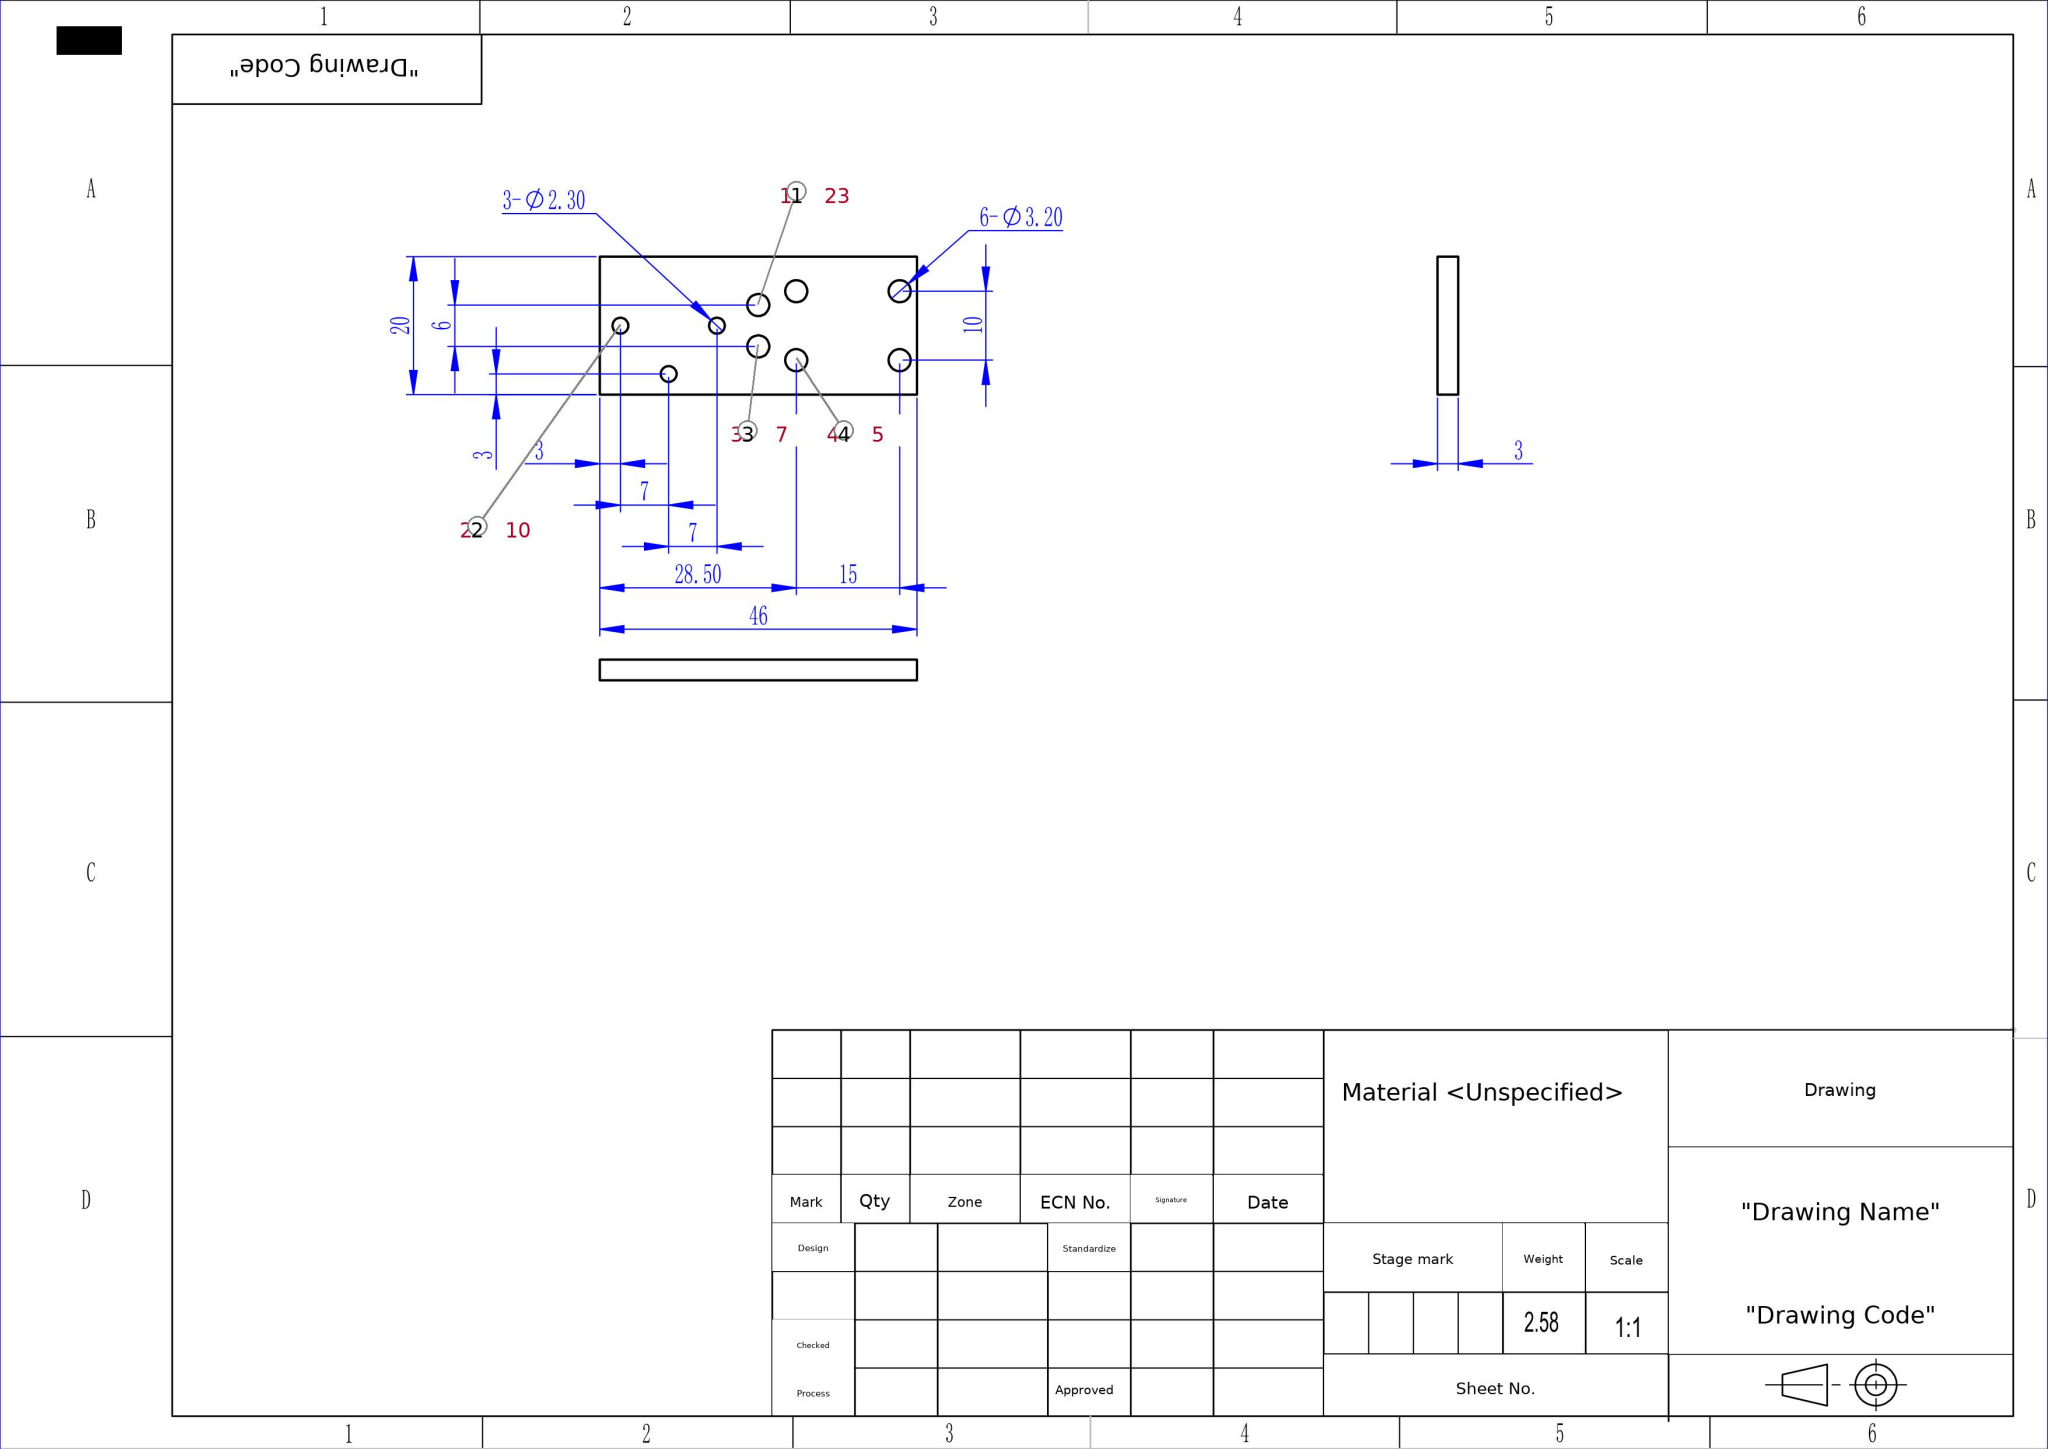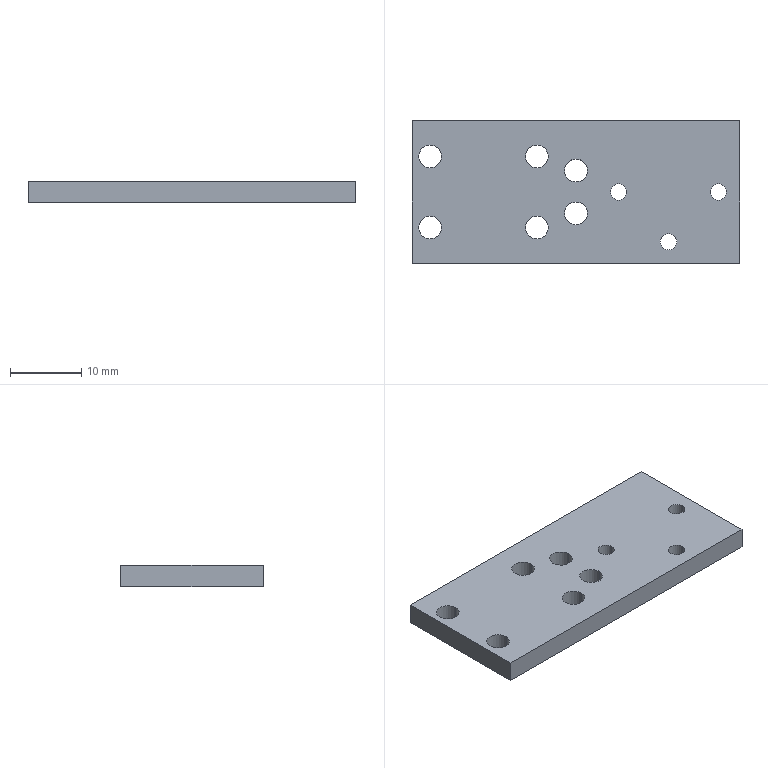Part | SolidWorks | mm | 1 solid | 24 faces | box 46 x 20 x 3 mm | volume 2578 mm3 | cylinder 18 | plane 6 | commonest cylinder face diameters 3.2 x12 2.3 x6
build123d program:
from build123d import *

# Parameters (mm, degrees)
SKETCH1_W           = 46
SKETCH1_H           = 20
SKETCH1_R           = 1.6
SKETCH1_R_2         = 1.15
BOSS_EXTRUDE1_DEPTH = 3


with BuildPart() as part:
    # Sketch1 → Boss-Extrude1 (new body)
    with BuildSketch(Plane.XY):
        with Locations((13, 0)):
            Rectangle(SKETCH1_W, SKETCH1_H)
        with Locations((-7.5, 5)):
            Circle(SKETCH1_R, mode=Mode.SUBTRACT)
        with Locations((7.5, 5)):
            Circle(SKETCH1_R, mode=Mode.SUBTRACT)
        with Locations((7.5, -5)):
            Circle(SKETCH1_R, mode=Mode.SUBTRACT)
        with Locations((-7.5, -5)):
            Circle(SKETCH1_R, mode=Mode.SUBTRACT)
        with Locations((26, -7)):
            Circle(SKETCH1_R_2, mode=Mode.SUBTRACT)
        with Locations((19, 0)):
            Circle(SKETCH1_R_2, mode=Mode.SUBTRACT)
        with Locations((33, 0)):
            Circle(SKETCH1_R_2, mode=Mode.SUBTRACT)
        with Locations((13, 3)):
            Circle(SKETCH1_R, mode=Mode.SUBTRACT)
        with Locations((13, -3)):
            Circle(SKETCH1_R, mode=Mode.SUBTRACT)
    extrude(amount=BOSS_EXTRUDE1_DEPTH)


solid = part.part
STEP:
#1=CARTESIAN_POINT('',(17.85,0.,3.));
#2=VERTEX_POINT('',#1);
#3=CARTESIAN_POINT('',(20.15,0.,3.));
#4=VERTEX_POINT('',#3);
#5=CARTESIAN_POINT('',(19.,0.,3.));
#6=DIRECTION('',(0.,0.,1.));
#7=DIRECTION('',(1.,0.,0.));
#8=AXIS2_PLACEMENT_3D('',#5,#6,#7);
#9=CIRCLE('',#8,1.15);
#10=EDGE_CURVE('',#2,#4,#9,.T.);
#11=ORIENTED_EDGE('',*,*,#10,.T.);
#12=CARTESIAN_POINT('',(20.15,0.,0.));
#13=VERTEX_POINT('',#12);
#14=CARTESIAN_POINT('',(20.15,0.,3.));
#15=DIRECTION('',(0.,0.,-1.));
#16=VECTOR('',#15,1000.);
#17=LINE('',#14,#16);
#18=EDGE_CURVE('',#4,#13,#17,.T.);
#19=ORIENTED_EDGE('',*,*,#18,.T.);
#20=CARTESIAN_POINT('',(17.85,0.,0.));
#21=VERTEX_POINT('',#20);
#22=CARTESIAN_POINT('',(19.,0.,0.));
#23=DIRECTION('',(0.,0.,1.));
#24=DIRECTION('',(1.,0.,0.));
#25=AXIS2_PLACEMENT_3D('',#22,#23,#24);
#26=CIRCLE('',#25,1.15);
#27=EDGE_CURVE('',#21,#13,#26,.T.);
#28=ORIENTED_EDGE('',*,*,#27,.F.);
#29=CARTESIAN_POINT('',(17.85,0.,3.));
#30=DIRECTION('',(0.,0.,-1.));
#31=VECTOR('',#30,1000.);
#32=LINE('',#29,#31);
#33=EDGE_CURVE('',#2,#21,#32,.T.);
#34=ORIENTED_EDGE('',*,*,#33,.F.);
#35=EDGE_LOOP('',(#11,#19,#28,#34));
#36=FACE_OUTER_BOUND('',#35,.T.);
#37=CARTESIAN_POINT('',(19.,0.,3.));
#38=DIRECTION('',(0.,0.,-1.));
#39=DIRECTION('',(-1.,0.,0.));
#40=AXIS2_PLACEMENT_3D('',#37,#38,#39);
#41=CYLINDRICAL_SURFACE('',#40,1.15);
#42=ADVANCED_FACE('',(#36),#41,.F.);
#43=CARTESIAN_POINT('',(24.85,-7.,3.));
#44=VERTEX_POINT('',#43);
#45=CARTESIAN_POINT('',(27.15,-7.,3.));
#46=VERTEX_POINT('',#45);
#47=CARTESIAN_POINT('',(26.,-7.,3.));
#48=DIRECTION('',(0.,0.,1.));
#49=DIRECTION('',(1.,0.,0.));
#50=AXIS2_PLACEMENT_3D('',#47,#48,#49);
#51=CIRCLE('',#50,1.15);
#52=EDGE_CURVE('',#44,#46,#51,.T.);
#53=ORIENTED_EDGE('',*,*,#52,.T.);
#54=CARTESIAN_POINT('',(27.15,-7.,0.));
#55=VERTEX_POINT('',#54);
#56=CARTESIAN_POINT('',(27.15,-7.,3.));
#57=DIRECTION('',(0.,0.,-1.));
#58=VECTOR('',#57,1000.);
#59=LINE('',#56,#58);
#60=EDGE_CURVE('',#46,#55,#59,.T.);
#61=ORIENTED_EDGE('',*,*,#60,.T.);
#62=CARTESIAN_POINT('',(24.85,-7.,0.));
#63=VERTEX_POINT('',#62);
#64=CARTESIAN_POINT('',(26.,-7.,0.));
#65=DIRECTION('',(0.,0.,1.));
#66=DIRECTION('',(1.,0.,0.));
#67=AXIS2_PLACEMENT_3D('',#64,#65,#66);
#68=CIRCLE('',#67,1.15);
#69=EDGE_CURVE('',#63,#55,#68,.T.);
#70=ORIENTED_EDGE('',*,*,#69,.F.);
#71=CARTESIAN_POINT('',(24.85,-7.,3.));
#72=DIRECTION('',(0.,0.,-1.));
#73=VECTOR('',#72,1000.);
#74=LINE('',#71,#73);
#75=EDGE_CURVE('',#44,#63,#74,.T.);
#76=ORIENTED_EDGE('',*,*,#75,.F.);
#77=EDGE_LOOP('',(#53,#61,#70,#76));
#78=FACE_OUTER_BOUND('',#77,.T.);
#79=CARTESIAN_POINT('',(26.,-7.,3.));
#80=DIRECTION('',(0.,0.,-1.));
#81=DIRECTION('',(-1.,0.,0.));
#82=AXIS2_PLACEMENT_3D('',#79,#80,#81);
#83=CYLINDRICAL_SURFACE('',#82,1.15);
#84=ADVANCED_FACE('',(#78),#83,.F.);
#85=CARTESIAN_POINT('',(11.4,-3.,3.));
#86=VERTEX_POINT('',#85);
#87=CARTESIAN_POINT('',(14.6,-3.,3.));
#88=VERTEX_POINT('',#87);
#89=CARTESIAN_POINT('',(13.,-3.,3.));
#90=DIRECTION('',(0.,0.,1.));
#91=DIRECTION('',(1.,0.,0.));
#92=AXIS2_PLACEMENT_3D('',#89,#90,#91);
#93=CIRCLE('',#92,1.6);
#94=EDGE_CURVE('',#86,#88,#93,.T.);
#95=ORIENTED_EDGE('',*,*,#94,.T.);
#96=CARTESIAN_POINT('',(14.6,-3.,0.));
#97=VERTEX_POINT('',#96);
#98=CARTESIAN_POINT('',(14.6,-3.,3.));
#99=DIRECTION('',(0.,0.,-1.));
#100=VECTOR('',#99,1000.);
#101=LINE('',#98,#100);
#102=EDGE_CURVE('',#88,#97,#101,.T.);
#103=ORIENTED_EDGE('',*,*,#102,.T.);
#104=CARTESIAN_POINT('',(11.4,-3.,0.));
#105=VERTEX_POINT('',#104);
#106=CARTESIAN_POINT('',(13.,-3.,0.));
#107=DIRECTION('',(0.,0.,1.));
#108=DIRECTION('',(1.,0.,0.));
#109=AXIS2_PLACEMENT_3D('',#106,#107,#108);
#110=CIRCLE('',#109,1.6);
#111=EDGE_CURVE('',#105,#97,#110,.T.);
#112=ORIENTED_EDGE('',*,*,#111,.F.);
#113=CARTESIAN_POINT('',(11.4,-3.,3.));
#114=DIRECTION('',(0.,0.,-1.));
#115=VECTOR('',#114,1000.);
#116=LINE('',#113,#115);
#117=EDGE_CURVE('',#86,#105,#116,.T.);
#118=ORIENTED_EDGE('',*,*,#117,.F.);
#119=EDGE_LOOP('',(#95,#103,#112,#118));
#120=FACE_OUTER_BOUND('',#119,.T.);
#121=CARTESIAN_POINT('',(13.,-3.,3.));
#122=DIRECTION('',(0.,0.,-1.));
#123=DIRECTION('',(-1.,0.,0.));
#124=AXIS2_PLACEMENT_3D('',#121,#122,#123);
#125=CYLINDRICAL_SURFACE('',#124,1.6);
#126=ADVANCED_FACE('',(#120),#125,.F.);
#127=CARTESIAN_POINT('',(31.85,0.,3.));
#128=VERTEX_POINT('',#127);
#129=CARTESIAN_POINT('',(34.15,0.,3.));
#130=VERTEX_POINT('',#129);
#131=CARTESIAN_POINT('',(33.,0.,3.));
#132=DIRECTION('',(0.,0.,1.));
#133=DIRECTION('',(1.,0.,0.));
#134=AXIS2_PLACEMENT_3D('',#131,#132,#133);
#135=CIRCLE('',#134,1.15);
#136=EDGE_CURVE('',#128,#130,#135,.T.);
#137=ORIENTED_EDGE('',*,*,#136,.T.);
#138=CARTESIAN_POINT('',(34.15,0.,0.));
#139=VERTEX_POINT('',#138);
#140=CARTESIAN_POINT('',(34.15,0.,3.));
#141=DIRECTION('',(0.,0.,-1.));
#142=VECTOR('',#141,1000.);
#143=LINE('',#140,#142);
#144=EDGE_CURVE('',#130,#139,#143,.T.);
#145=ORIENTED_EDGE('',*,*,#144,.T.);
#146=CARTESIAN_POINT('',(31.85,0.,0.));
#147=VERTEX_POINT('',#146);
#148=CARTESIAN_POINT('',(33.,0.,0.));
#149=DIRECTION('',(0.,0.,1.));
#150=DIRECTION('',(1.,0.,0.));
#151=AXIS2_PLACEMENT_3D('',#148,#149,#150);
#152=CIRCLE('',#151,1.15);
#153=EDGE_CURVE('',#147,#139,#152,.T.);
#154=ORIENTED_EDGE('',*,*,#153,.F.);
#155=CARTESIAN_POINT('',(31.85,0.,3.));
#156=DIRECTION('',(0.,0.,-1.));
#157=VECTOR('',#156,1000.);
#158=LINE('',#155,#157);
#159=EDGE_CURVE('',#128,#147,#158,.T.);
#160=ORIENTED_EDGE('',*,*,#159,.F.);
#161=EDGE_LOOP('',(#137,#145,#154,#160));
#162=FACE_OUTER_BOUND('',#161,.T.);
#163=CARTESIAN_POINT('',(33.,0.,3.));
#164=DIRECTION('',(0.,0.,-1.));
#165=DIRECTION('',(-1.,0.,0.));
#166=AXIS2_PLACEMENT_3D('',#163,#164,#165);
#167=CYLINDRICAL_SURFACE('',#166,1.15);
#168=ADVANCED_FACE('',(#162),#167,.F.);
#169=CARTESIAN_POINT('',(11.4,3.,3.));
#170=VERTEX_POINT('',#169);
#171=CARTESIAN_POINT('',(14.6,3.,3.));
#172=VERTEX_POINT('',#171);
#173=CARTESIAN_POINT('',(13.,3.,3.));
#174=DIRECTION('',(0.,0.,1.));
#175=DIRECTION('',(1.,0.,0.));
#176=AXIS2_PLACEMENT_3D('',#173,#174,#175);
#177=CIRCLE('',#176,1.6);
#178=EDGE_CURVE('',#170,#172,#177,.T.);
#179=ORIENTED_EDGE('',*,*,#178,.T.);
#180=CARTESIAN_POINT('',(14.6,3.,0.));
#181=VERTEX_POINT('',#180);
#182=CARTESIAN_POINT('',(14.6,3.,3.));
#183=DIRECTION('',(0.,0.,-1.));
#184=VECTOR('',#183,1000.);
#185=LINE('',#182,#184);
#186=EDGE_CURVE('',#172,#181,#185,.T.);
#187=ORIENTED_EDGE('',*,*,#186,.T.);
#188=CARTESIAN_POINT('',(11.4,3.,0.));
#189=VERTEX_POINT('',#188);
#190=CARTESIAN_POINT('',(13.,3.,0.));
#191=DIRECTION('',(0.,0.,1.));
#192=DIRECTION('',(1.,0.,0.));
#193=AXIS2_PLACEMENT_3D('',#190,#191,#192);
#194=CIRCLE('',#193,1.6);
#195=EDGE_CURVE('',#189,#181,#194,.T.);
#196=ORIENTED_EDGE('',*,*,#195,.F.);
#197=CARTESIAN_POINT('',(11.4,3.,3.));
#198=DIRECTION('',(0.,0.,-1.));
#199=VECTOR('',#198,1000.);
#200=LINE('',#197,#199);
#201=EDGE_CURVE('',#170,#189,#200,.T.);
#202=ORIENTED_EDGE('',*,*,#201,.F.);
#203=EDGE_LOOP('',(#179,#187,#196,#202));
#204=FACE_OUTER_BOUND('',#203,.T.);
#205=CARTESIAN_POINT('',(13.,3.,3.));
#206=DIRECTION('',(0.,0.,-1.));
#207=DIRECTION('',(-1.,0.,0.));
#208=AXIS2_PLACEMENT_3D('',#205,#206,#207);
#209=CYLINDRICAL_SURFACE('',#208,1.6);
#210=ADVANCED_FACE('',(#204),#209,.F.);
#211=CARTESIAN_POINT('',(-9.1,-5.,3.));
#212=VERTEX_POINT('',#211);
#213=CARTESIAN_POINT('',(-5.9,-5.,3.));
#214=VERTEX_POINT('',#213);
#215=CARTESIAN_POINT('',(-7.5,-5.,3.));
#216=DIRECTION('',(0.,0.,1.));
#217=DIRECTION('',(1.,0.,0.));
#218=AXIS2_PLACEMENT_3D('',#215,#216,#217);
#219=CIRCLE('',#218,1.6);
#220=EDGE_CURVE('',#212,#214,#219,.T.);
#221=ORIENTED_EDGE('',*,*,#220,.T.);
#222=CARTESIAN_POINT('',(-5.9,-5.,0.));
#223=VERTEX_POINT('',#222);
#224=CARTESIAN_POINT('',(-5.9,-5.,3.));
#225=DIRECTION('',(0.,0.,-1.));
#226=VECTOR('',#225,1000.);
#227=LINE('',#224,#226);
#228=EDGE_CURVE('',#214,#223,#227,.T.);
#229=ORIENTED_EDGE('',*,*,#228,.T.);
#230=CARTESIAN_POINT('',(-9.1,-5.,0.));
#231=VERTEX_POINT('',#230);
#232=CARTESIAN_POINT('',(-7.5,-5.,0.));
#233=DIRECTION('',(0.,0.,1.));
#234=DIRECTION('',(1.,0.,0.));
#235=AXIS2_PLACEMENT_3D('',#232,#233,#234);
#236=CIRCLE('',#235,1.6);
#237=EDGE_CURVE('',#231,#223,#236,.T.);
#238=ORIENTED_EDGE('',*,*,#237,.F.);
#239=CARTESIAN_POINT('',(-9.1,-5.,3.));
#240=DIRECTION('',(0.,0.,-1.));
#241=VECTOR('',#240,1000.);
#242=LINE('',#239,#241);
#243=EDGE_CURVE('',#212,#231,#242,.T.);
#244=ORIENTED_EDGE('',*,*,#243,.F.);
#245=EDGE_LOOP('',(#221,#229,#238,#244));
#246=FACE_OUTER_BOUND('',#245,.T.);
#247=CARTESIAN_POINT('',(-7.5,-5.,3.));
#248=DIRECTION('',(0.,0.,-1.));
#249=DIRECTION('',(-1.,0.,0.));
#250=AXIS2_PLACEMENT_3D('',#247,#248,#249);
#251=CYLINDRICAL_SURFACE('',#250,1.6);
#252=ADVANCED_FACE('',(#246),#251,.F.);
#253=CARTESIAN_POINT('',(5.9,-5.,3.));
#254=VERTEX_POINT('',#253);
#255=CARTESIAN_POINT('',(9.1,-5.,3.));
#256=VERTEX_POINT('',#255);
#257=CARTESIAN_POINT('',(7.5,-5.,3.));
#258=DIRECTION('',(0.,0.,1.));
#259=DIRECTION('',(1.,0.,0.));
#260=AXIS2_PLACEMENT_3D('',#257,#258,#259);
#261=CIRCLE('',#260,1.6);
#262=EDGE_CURVE('',#254,#256,#261,.T.);
#263=ORIENTED_EDGE('',*,*,#262,.T.);
#264=CARTESIAN_POINT('',(9.1,-5.,0.));
#265=VERTEX_POINT('',#264);
#266=CARTESIAN_POINT('',(9.1,-5.,3.));
#267=DIRECTION('',(0.,0.,-1.));
#268=VECTOR('',#267,1000.);
#269=LINE('',#266,#268);
#270=EDGE_CURVE('',#256,#265,#269,.T.);
#271=ORIENTED_EDGE('',*,*,#270,.T.);
#272=CARTESIAN_POINT('',(5.9,-5.,0.));
#273=VERTEX_POINT('',#272);
#274=CARTESIAN_POINT('',(7.5,-5.,0.));
#275=DIRECTION('',(0.,0.,1.));
#276=DIRECTION('',(1.,0.,0.));
#277=AXIS2_PLACEMENT_3D('',#274,#275,#276);
#278=CIRCLE('',#277,1.6);
#279=EDGE_CURVE('',#273,#265,#278,.T.);
#280=ORIENTED_EDGE('',*,*,#279,.F.);
#281=CARTESIAN_POINT('',(5.9,-5.,3.));
#282=DIRECTION('',(0.,0.,-1.));
#283=VECTOR('',#282,1000.);
#284=LINE('',#281,#283);
#285=EDGE_CURVE('',#254,#273,#284,.T.);
#286=ORIENTED_EDGE('',*,*,#285,.F.);
#287=EDGE_LOOP('',(#263,#271,#280,#286));
#288=FACE_OUTER_BOUND('',#287,.T.);
#289=CARTESIAN_POINT('',(7.5,-5.,3.));
#290=DIRECTION('',(0.,0.,-1.));
#291=DIRECTION('',(-1.,0.,0.));
#292=AXIS2_PLACEMENT_3D('',#289,#290,#291);
#293=CYLINDRICAL_SURFACE('',#292,1.6);
#294=ADVANCED_FACE('',(#288),#293,.F.);
#295=CARTESIAN_POINT('',(-9.1,5.,3.));
#296=VERTEX_POINT('',#295);
#297=CARTESIAN_POINT('',(-5.9,5.,3.));
#298=VERTEX_POINT('',#297);
#299=CARTESIAN_POINT('',(-7.5,5.,3.));
#300=DIRECTION('',(0.,0.,1.));
#301=DIRECTION('',(1.,0.,0.));
#302=AXIS2_PLACEMENT_3D('',#299,#300,#301);
#303=CIRCLE('',#302,1.6);
#304=EDGE_CURVE('',#296,#298,#303,.T.);
#305=ORIENTED_EDGE('',*,*,#304,.T.);
#306=CARTESIAN_POINT('',(-5.9,5.,0.));
#307=VERTEX_POINT('',#306);
#308=CARTESIAN_POINT('',(-5.9,5.,3.));
#309=DIRECTION('',(0.,0.,-1.));
#310=VECTOR('',#309,1000.);
#311=LINE('',#308,#310);
#312=EDGE_CURVE('',#298,#307,#311,.T.);
#313=ORIENTED_EDGE('',*,*,#312,.T.);
#314=CARTESIAN_POINT('',(-9.1,5.,0.));
#315=VERTEX_POINT('',#314);
#316=CARTESIAN_POINT('',(-7.5,5.,0.));
#317=DIRECTION('',(0.,0.,1.));
#318=DIRECTION('',(1.,0.,0.));
#319=AXIS2_PLACEMENT_3D('',#316,#317,#318);
#320=CIRCLE('',#319,1.6);
#321=EDGE_CURVE('',#315,#307,#320,.T.);
#322=ORIENTED_EDGE('',*,*,#321,.F.);
#323=CARTESIAN_POINT('',(-9.1,5.,3.));
#324=DIRECTION('',(0.,0.,-1.));
#325=VECTOR('',#324,1000.);
#326=LINE('',#323,#325);
#327=EDGE_CURVE('',#296,#315,#326,.T.);
#328=ORIENTED_EDGE('',*,*,#327,.F.);
#329=EDGE_LOOP('',(#305,#313,#322,#328));
#330=FACE_OUTER_BOUND('',#329,.T.);
#331=CARTESIAN_POINT('',(-7.5,5.,3.));
#332=DIRECTION('',(0.,0.,-1.));
#333=DIRECTION('',(-1.,0.,0.));
#334=AXIS2_PLACEMENT_3D('',#331,#332,#333);
#335=CYLINDRICAL_SURFACE('',#334,1.6);
#336=ADVANCED_FACE('',(#330),#335,.F.);
#337=CARTESIAN_POINT('',(5.9,5.,3.));
#338=VERTEX_POINT('',#337);
#339=CARTESIAN_POINT('',(9.1,5.,3.));
#340=VERTEX_POINT('',#339);
#341=CARTESIAN_POINT('',(7.5,5.,3.));
#342=DIRECTION('',(0.,0.,1.));
#343=DIRECTION('',(1.,0.,0.));
#344=AXIS2_PLACEMENT_3D('',#341,#342,#343);
#345=CIRCLE('',#344,1.6);
#346=EDGE_CURVE('',#338,#340,#345,.T.);
#347=ORIENTED_EDGE('',*,*,#346,.T.);
#348=CARTESIAN_POINT('',(9.1,5.,0.));
#349=VERTEX_POINT('',#348);
#350=CARTESIAN_POINT('',(9.1,5.,3.));
#351=DIRECTION('',(0.,0.,-1.));
#352=VECTOR('',#351,1000.);
#353=LINE('',#350,#352);
#354=EDGE_CURVE('',#340,#349,#353,.T.);
#355=ORIENTED_EDGE('',*,*,#354,.T.);
#356=CARTESIAN_POINT('',(5.9,5.,0.));
#357=VERTEX_POINT('',#356);
#358=CARTESIAN_POINT('',(7.5,5.,0.));
#359=DIRECTION('',(0.,0.,1.));
#360=DIRECTION('',(1.,0.,0.));
#361=AXIS2_PLACEMENT_3D('',#358,#359,#360);
#362=CIRCLE('',#361,1.6);
#363=EDGE_CURVE('',#357,#349,#362,.T.);
#364=ORIENTED_EDGE('',*,*,#363,.F.);
#365=CARTESIAN_POINT('',(5.9,5.,3.));
#366=DIRECTION('',(0.,0.,-1.));
#367=VECTOR('',#366,1000.);
#368=LINE('',#365,#367);
#369=EDGE_CURVE('',#338,#357,#368,.T.);
#370=ORIENTED_EDGE('',*,*,#369,.F.);
#371=EDGE_LOOP('',(#347,#355,#364,#370));
#372=FACE_OUTER_BOUND('',#371,.T.);
#373=CARTESIAN_POINT('',(7.5,5.,3.));
#374=DIRECTION('',(0.,0.,-1.));
#375=DIRECTION('',(-1.,0.,0.));
#376=AXIS2_PLACEMENT_3D('',#373,#374,#375);
#377=CYLINDRICAL_SURFACE('',#376,1.6);
#378=ADVANCED_FACE('',(#372),#377,.F.);
#379=ORIENTED_EDGE('',*,*,#52,.F.);
#380=CARTESIAN_POINT('',(26.,-7.,3.));
#381=DIRECTION('',(0.,0.,1.));
#382=DIRECTION('',(1.,0.,0.));
#383=AXIS2_PLACEMENT_3D('',#380,#381,#382);
#384=CIRCLE('',#383,1.15);
#385=EDGE_CURVE('',#46,#44,#384,.T.);
#386=ORIENTED_EDGE('',*,*,#385,.F.);
#387=EDGE_LOOP('',(#379,#386));
#388=FACE_BOUND('',#387,.T.);
#389=ORIENTED_EDGE('',*,*,#136,.F.);
#390=CARTESIAN_POINT('',(33.,0.,3.));
#391=DIRECTION('',(0.,0.,1.));
#392=DIRECTION('',(1.,0.,0.));
#393=AXIS2_PLACEMENT_3D('',#390,#391,#392);
#394=CIRCLE('',#393,1.15);
#395=EDGE_CURVE('',#130,#128,#394,.T.);
#396=ORIENTED_EDGE('',*,*,#395,.F.);
#397=EDGE_LOOP('',(#389,#396));
#398=FACE_BOUND('',#397,.T.);
#399=ORIENTED_EDGE('',*,*,#220,.F.);
#400=CARTESIAN_POINT('',(-7.5,-5.,3.));
#401=DIRECTION('',(0.,0.,1.));
#402=DIRECTION('',(1.,0.,0.));
#403=AXIS2_PLACEMENT_3D('',#400,#401,#402);
#404=CIRCLE('',#403,1.6);
#405=EDGE_CURVE('',#214,#212,#404,.T.);
#406=ORIENTED_EDGE('',*,*,#405,.F.);
#407=EDGE_LOOP('',(#399,#406));
#408=FACE_BOUND('',#407,.T.);
#409=ORIENTED_EDGE('',*,*,#304,.F.);
#410=CARTESIAN_POINT('',(-7.5,5.,3.));
#411=DIRECTION('',(0.,0.,1.));
#412=DIRECTION('',(1.,0.,0.));
#413=AXIS2_PLACEMENT_3D('',#410,#411,#412);
#414=CIRCLE('',#413,1.6);
#415=EDGE_CURVE('',#298,#296,#414,.T.);
#416=ORIENTED_EDGE('',*,*,#415,.F.);
#417=EDGE_LOOP('',(#409,#416));
#418=FACE_BOUND('',#417,.T.);
#419=CARTESIAN_POINT('',(-10.,10.,3.));
#420=VERTEX_POINT('',#419);
#421=CARTESIAN_POINT('',(-10.,-10.,3.));
#422=VERTEX_POINT('',#421);
#423=CARTESIAN_POINT('',(-10.,10.,3.));
#424=DIRECTION('',(0.,-1.,0.));
#425=VECTOR('',#424,1000.);
#426=LINE('',#423,#425);
#427=EDGE_CURVE('',#420,#422,#426,.T.);
#428=ORIENTED_EDGE('',*,*,#427,.T.);
#429=CARTESIAN_POINT('',(36.,-10.,3.));
#430=VERTEX_POINT('',#429);
#431=CARTESIAN_POINT('',(-10.,-10.,3.));
#432=DIRECTION('',(1.,0.,0.));
#433=VECTOR('',#432,1000.);
#434=LINE('',#431,#433);
#435=EDGE_CURVE('',#422,#430,#434,.T.);
#436=ORIENTED_EDGE('',*,*,#435,.T.);
#437=CARTESIAN_POINT('',(36.,10.,3.));
#438=VERTEX_POINT('',#437);
#439=CARTESIAN_POINT('',(36.,10.,3.));
#440=DIRECTION('',(0.,1.,0.));
#441=VECTOR('',#440,1000.);
#442=LINE('',#439,#441);
#443=EDGE_CURVE('',#430,#438,#442,.T.);
#444=ORIENTED_EDGE('',*,*,#443,.T.);
#445=CARTESIAN_POINT('',(-10.,10.,3.));
#446=DIRECTION('',(-1.,0.,0.));
#447=VECTOR('',#446,1000.);
#448=LINE('',#445,#447);
#449=EDGE_CURVE('',#438,#420,#448,.T.);
#450=ORIENTED_EDGE('',*,*,#449,.T.);
#451=EDGE_LOOP('',(#428,#436,#444,#450));
#452=FACE_OUTER_BOUND('',#451,.T.);
#453=ORIENTED_EDGE('',*,*,#346,.F.);
#454=CARTESIAN_POINT('',(7.5,5.,3.));
#455=DIRECTION('',(0.,0.,1.));
#456=DIRECTION('',(1.,0.,0.));
#457=AXIS2_PLACEMENT_3D('',#454,#455,#456);
#458=CIRCLE('',#457,1.6);
#459=EDGE_CURVE('',#340,#338,#458,.T.);
#460=ORIENTED_EDGE('',*,*,#459,.F.);
#461=EDGE_LOOP('',(#453,#460));
#462=FACE_BOUND('',#461,.T.);
#463=ORIENTED_EDGE('',*,*,#262,.F.);
#464=CARTESIAN_POINT('',(7.5,-5.,3.));
#465=DIRECTION('',(0.,0.,1.));
#466=DIRECTION('',(1.,0.,0.));
#467=AXIS2_PLACEMENT_3D('',#464,#465,#466);
#468=CIRCLE('',#467,1.6);
#469=EDGE_CURVE('',#256,#254,#468,.T.);
#470=ORIENTED_EDGE('',*,*,#469,.F.);
#471=EDGE_LOOP('',(#463,#470));
#472=FACE_BOUND('',#471,.T.);
#473=ORIENTED_EDGE('',*,*,#178,.F.);
#474=CARTESIAN_POINT('',(13.,3.,3.));
#475=DIRECTION('',(0.,0.,1.));
#476=DIRECTION('',(1.,0.,0.));
#477=AXIS2_PLACEMENT_3D('',#474,#475,#476);
#478=CIRCLE('',#477,1.6);
#479=EDGE_CURVE('',#172,#170,#478,.T.);
#480=ORIENTED_EDGE('',*,*,#479,.F.);
#481=EDGE_LOOP('',(#473,#480));
#482=FACE_BOUND('',#481,.T.);
#483=ORIENTED_EDGE('',*,*,#94,.F.);
#484=CARTESIAN_POINT('',(13.,-3.,3.));
#485=DIRECTION('',(0.,0.,1.));
#486=DIRECTION('',(1.,0.,0.));
#487=AXIS2_PLACEMENT_3D('',#484,#485,#486);
#488=CIRCLE('',#487,1.6);
#489=EDGE_CURVE('',#88,#86,#488,.T.);
#490=ORIENTED_EDGE('',*,*,#489,.F.);
#491=EDGE_LOOP('',(#483,#490));
#492=FACE_BOUND('',#491,.T.);
#493=ORIENTED_EDGE('',*,*,#10,.F.);
#494=CARTESIAN_POINT('',(19.,0.,3.));
#495=DIRECTION('',(0.,0.,1.));
#496=DIRECTION('',(1.,0.,0.));
#497=AXIS2_PLACEMENT_3D('',#494,#495,#496);
#498=CIRCLE('',#497,1.15);
#499=EDGE_CURVE('',#4,#2,#498,.T.);
#500=ORIENTED_EDGE('',*,*,#499,.F.);
#501=EDGE_LOOP('',(#493,#500));
#502=FACE_BOUND('',#501,.T.);
#503=CARTESIAN_POINT('',(0.,0.,3.));
#504=DIRECTION('',(0.,0.,1.));
#505=DIRECTION('',(1.,0.,0.));
#506=AXIS2_PLACEMENT_3D('',#503,#504,#505);
#507=PLANE('',#506);
#508=ADVANCED_FACE('',(#388,#398,#408,#418,#452,#462,#472,#482,#492,#502),#507,.T.);
#509=CARTESIAN_POINT('',(-10.,10.,0.));
#510=VERTEX_POINT('',#509);
#511=CARTESIAN_POINT('',(-10.,-10.,0.));
#512=VERTEX_POINT('',#511);
#513=CARTESIAN_POINT('',(-10.,10.,0.));
#514=DIRECTION('',(0.,-1.,0.));
#515=VECTOR('',#514,1000.);
#516=LINE('',#513,#515);
#517=EDGE_CURVE('',#510,#512,#516,.T.);
#518=ORIENTED_EDGE('',*,*,#517,.F.);
#519=CARTESIAN_POINT('',(36.,10.,0.));
#520=VERTEX_POINT('',#519);
#521=CARTESIAN_POINT('',(-10.,10.,0.));
#522=DIRECTION('',(-1.,0.,0.));
#523=VECTOR('',#522,1000.);
#524=LINE('',#521,#523);
#525=EDGE_CURVE('',#520,#510,#524,.T.);
#526=ORIENTED_EDGE('',*,*,#525,.F.);
#527=CARTESIAN_POINT('',(36.,-10.,0.));
#528=VERTEX_POINT('',#527);
#529=CARTESIAN_POINT('',(36.,10.,0.));
#530=DIRECTION('',(0.,1.,0.));
#531=VECTOR('',#530,1000.);
#532=LINE('',#529,#531);
#533=EDGE_CURVE('',#528,#520,#532,.T.);
#534=ORIENTED_EDGE('',*,*,#533,.F.);
#535=CARTESIAN_POINT('',(-10.,-10.,0.));
#536=DIRECTION('',(1.,0.,0.));
#537=VECTOR('',#536,1000.);
#538=LINE('',#535,#537);
#539=EDGE_CURVE('',#512,#528,#538,.T.);
#540=ORIENTED_EDGE('',*,*,#539,.F.);
#541=EDGE_LOOP('',(#518,#526,#534,#540));
#542=FACE_OUTER_BOUND('',#541,.T.);
#543=ORIENTED_EDGE('',*,*,#363,.T.);
#544=CARTESIAN_POINT('',(7.5,5.,0.));
#545=DIRECTION('',(0.,0.,1.));
#546=DIRECTION('',(1.,0.,0.));
#547=AXIS2_PLACEMENT_3D('',#544,#545,#546);
#548=CIRCLE('',#547,1.6);
#549=EDGE_CURVE('',#349,#357,#548,.T.);
#550=ORIENTED_EDGE('',*,*,#549,.T.);
#551=EDGE_LOOP('',(#543,#550));
#552=FACE_BOUND('',#551,.T.);
#553=ORIENTED_EDGE('',*,*,#321,.T.);
#554=CARTESIAN_POINT('',(-7.5,5.,0.));
#555=DIRECTION('',(0.,0.,1.));
#556=DIRECTION('',(1.,0.,0.));
#557=AXIS2_PLACEMENT_3D('',#554,#555,#556);
#558=CIRCLE('',#557,1.6);
#559=EDGE_CURVE('',#307,#315,#558,.T.);
#560=ORIENTED_EDGE('',*,*,#559,.T.);
#561=EDGE_LOOP('',(#553,#560));
#562=FACE_BOUND('',#561,.T.);
#563=ORIENTED_EDGE('',*,*,#279,.T.);
#564=CARTESIAN_POINT('',(7.5,-5.,0.));
#565=DIRECTION('',(0.,0.,1.));
#566=DIRECTION('',(1.,0.,0.));
#567=AXIS2_PLACEMENT_3D('',#564,#565,#566);
#568=CIRCLE('',#567,1.6);
#569=EDGE_CURVE('',#265,#273,#568,.T.);
#570=ORIENTED_EDGE('',*,*,#569,.T.);
#571=EDGE_LOOP('',(#563,#570));
#572=FACE_BOUND('',#571,.T.);
#573=ORIENTED_EDGE('',*,*,#237,.T.);
#574=CARTESIAN_POINT('',(-7.5,-5.,0.));
#575=DIRECTION('',(0.,0.,1.));
#576=DIRECTION('',(1.,0.,0.));
#577=AXIS2_PLACEMENT_3D('',#574,#575,#576);
#578=CIRCLE('',#577,1.6);
#579=EDGE_CURVE('',#223,#231,#578,.T.);
#580=ORIENTED_EDGE('',*,*,#579,.T.);
#581=EDGE_LOOP('',(#573,#580));
#582=FACE_BOUND('',#581,.T.);
#583=ORIENTED_EDGE('',*,*,#195,.T.);
#584=CARTESIAN_POINT('',(13.,3.,0.));
#585=DIRECTION('',(0.,0.,1.));
#586=DIRECTION('',(1.,0.,0.));
#587=AXIS2_PLACEMENT_3D('',#584,#585,#586);
#588=CIRCLE('',#587,1.6);
#589=EDGE_CURVE('',#181,#189,#588,.T.);
#590=ORIENTED_EDGE('',*,*,#589,.T.);
#591=EDGE_LOOP('',(#583,#590));
#592=FACE_BOUND('',#591,.T.);
#593=ORIENTED_EDGE('',*,*,#153,.T.);
#594=CARTESIAN_POINT('',(33.,0.,0.));
#595=DIRECTION('',(0.,0.,1.));
#596=DIRECTION('',(1.,0.,0.));
#597=AXIS2_PLACEMENT_3D('',#594,#595,#596);
#598=CIRCLE('',#597,1.15);
#599=EDGE_CURVE('',#139,#147,#598,.T.);
#600=ORIENTED_EDGE('',*,*,#599,.T.);
#601=EDGE_LOOP('',(#593,#600));
#602=FACE_BOUND('',#601,.T.);
#603=ORIENTED_EDGE('',*,*,#111,.T.);
#604=CARTESIAN_POINT('',(13.,-3.,0.));
#605=DIRECTION('',(0.,0.,1.));
#606=DIRECTION('',(1.,0.,0.));
#607=AXIS2_PLACEMENT_3D('',#604,#605,#606);
#608=CIRCLE('',#607,1.6);
#609=EDGE_CURVE('',#97,#105,#608,.T.);
#610=ORIENTED_EDGE('',*,*,#609,.T.);
#611=EDGE_LOOP('',(#603,#610));
#612=FACE_BOUND('',#611,.T.);
#613=ORIENTED_EDGE('',*,*,#69,.T.);
#614=CARTESIAN_POINT('',(26.,-7.,0.));
#615=DIRECTION('',(0.,0.,1.));
#616=DIRECTION('',(1.,0.,0.));
#617=AXIS2_PLACEMENT_3D('',#614,#615,#616);
#618=CIRCLE('',#617,1.15);
#619=EDGE_CURVE('',#55,#63,#618,.T.);
#620=ORIENTED_EDGE('',*,*,#619,.T.);
#621=EDGE_LOOP('',(#613,#620));
#622=FACE_BOUND('',#621,.T.);
#623=ORIENTED_EDGE('',*,*,#27,.T.);
#624=CARTESIAN_POINT('',(19.,0.,0.));
#625=DIRECTION('',(0.,0.,1.));
#626=DIRECTION('',(1.,0.,0.));
#627=AXIS2_PLACEMENT_3D('',#624,#625,#626);
#628=CIRCLE('',#627,1.15);
#629=EDGE_CURVE('',#13,#21,#628,.T.);
#630=ORIENTED_EDGE('',*,*,#629,.T.);
#631=EDGE_LOOP('',(#623,#630));
#632=FACE_BOUND('',#631,.T.);
#633=CARTESIAN_POINT('',(0.,0.,0.));
#634=DIRECTION('',(0.,0.,1.));
#635=DIRECTION('',(1.,0.,0.));
#636=AXIS2_PLACEMENT_3D('',#633,#634,#635);
#637=PLANE('',#636);
#638=ADVANCED_FACE('',(#542,#552,#562,#572,#582,#592,#602,#612,#622,#632),#637,.F.);
#639=ORIENTED_EDGE('',*,*,#517,.T.);
#640=CARTESIAN_POINT('',(-10.,-10.,3.));
#641=DIRECTION('',(0.,0.,-1.));
#642=VECTOR('',#641,1000.);
#643=LINE('',#640,#642);
#644=EDGE_CURVE('',#422,#512,#643,.T.);
#645=ORIENTED_EDGE('',*,*,#644,.F.);
#646=ORIENTED_EDGE('',*,*,#427,.F.);
#647=CARTESIAN_POINT('',(-10.,10.,3.));
#648=DIRECTION('',(0.,0.,-1.));
#649=VECTOR('',#648,1000.);
#650=LINE('',#647,#649);
#651=EDGE_CURVE('',#420,#510,#650,.T.);
#652=ORIENTED_EDGE('',*,*,#651,.T.);
#653=EDGE_LOOP('',(#639,#645,#646,#652));
#654=FACE_OUTER_BOUND('',#653,.T.);
#655=CARTESIAN_POINT('',(-10.,10.,3.));
#656=DIRECTION('',(1.,0.,0.));
#657=DIRECTION('',(0.,0.,-1.));
#658=AXIS2_PLACEMENT_3D('',#655,#656,#657);
#659=PLANE('',#658);
#660=ADVANCED_FACE('',(#654),#659,.F.);
#661=ORIENTED_EDGE('',*,*,#539,.T.);
#662=CARTESIAN_POINT('',(36.,-10.,3.));
#663=DIRECTION('',(0.,0.,-1.));
#664=VECTOR('',#663,1000.);
#665=LINE('',#662,#664);
#666=EDGE_CURVE('',#430,#528,#665,.T.);
#667=ORIENTED_EDGE('',*,*,#666,.F.);
#668=ORIENTED_EDGE('',*,*,#435,.F.);
#669=ORIENTED_EDGE('',*,*,#644,.T.);
#670=EDGE_LOOP('',(#661,#667,#668,#669));
#671=FACE_OUTER_BOUND('',#670,.T.);
#672=CARTESIAN_POINT('',(-10.,-10.,3.));
#673=DIRECTION('',(-0.,1.,0.));
#674=DIRECTION('',(-1.,-0.,0.));
#675=AXIS2_PLACEMENT_3D('',#672,#673,#674);
#676=PLANE('',#675);
#677=ADVANCED_FACE('',(#671),#676,.F.);
#678=ORIENTED_EDGE('',*,*,#533,.T.);
#679=CARTESIAN_POINT('',(36.,10.,3.));
#680=DIRECTION('',(0.,0.,-1.));
#681=VECTOR('',#680,1000.);
#682=LINE('',#679,#681);
#683=EDGE_CURVE('',#438,#520,#682,.T.);
#684=ORIENTED_EDGE('',*,*,#683,.F.);
#685=ORIENTED_EDGE('',*,*,#443,.F.);
#686=ORIENTED_EDGE('',*,*,#666,.T.);
#687=EDGE_LOOP('',(#678,#684,#685,#686));
#688=FACE_OUTER_BOUND('',#687,.T.);
#689=CARTESIAN_POINT('',(36.,10.,3.));
#690=DIRECTION('',(-1.,0.,0.));
#691=DIRECTION('',(0.,0.,1.));
#692=AXIS2_PLACEMENT_3D('',#689,#690,#691);
#693=PLANE('',#692);
#694=ADVANCED_FACE('',(#688),#693,.F.);
#695=ORIENTED_EDGE('',*,*,#525,.T.);
#696=ORIENTED_EDGE('',*,*,#651,.F.);
#697=ORIENTED_EDGE('',*,*,#449,.F.);
#698=ORIENTED_EDGE('',*,*,#683,.T.);
#699=EDGE_LOOP('',(#695,#696,#697,#698));
#700=FACE_OUTER_BOUND('',#699,.T.);
#701=CARTESIAN_POINT('',(-10.,10.,3.));
#702=DIRECTION('',(-0.,-1.,0.));
#703=DIRECTION('',(1.,-0.,0.));
#704=AXIS2_PLACEMENT_3D('',#701,#702,#703);
#705=PLANE('',#704);
#706=ADVANCED_FACE('',(#700),#705,.F.);
#707=ORIENTED_EDGE('',*,*,#354,.F.);
#708=ORIENTED_EDGE('',*,*,#459,.T.);
#709=ORIENTED_EDGE('',*,*,#369,.T.);
#710=ORIENTED_EDGE('',*,*,#549,.F.);
#711=EDGE_LOOP('',(#707,#708,#709,#710));
#712=FACE_OUTER_BOUND('',#711,.T.);
#713=CARTESIAN_POINT('',(7.5,5.,3.));
#714=DIRECTION('',(0.,0.,-1.));
#715=DIRECTION('',(-1.,0.,0.));
#716=AXIS2_PLACEMENT_3D('',#713,#714,#715);
#717=CYLINDRICAL_SURFACE('',#716,1.6);
#718=ADVANCED_FACE('',(#712),#717,.F.);
#719=ORIENTED_EDGE('',*,*,#312,.F.);
#720=ORIENTED_EDGE('',*,*,#415,.T.);
#721=ORIENTED_EDGE('',*,*,#327,.T.);
#722=ORIENTED_EDGE('',*,*,#559,.F.);
#723=EDGE_LOOP('',(#719,#720,#721,#722));
#724=FACE_OUTER_BOUND('',#723,.T.);
#725=CARTESIAN_POINT('',(-7.5,5.,3.));
#726=DIRECTION('',(0.,0.,-1.));
#727=DIRECTION('',(-1.,0.,0.));
#728=AXIS2_PLACEMENT_3D('',#725,#726,#727);
#729=CYLINDRICAL_SURFACE('',#728,1.6);
#730=ADVANCED_FACE('',(#724),#729,.F.);
#731=ORIENTED_EDGE('',*,*,#270,.F.);
#732=ORIENTED_EDGE('',*,*,#469,.T.);
#733=ORIENTED_EDGE('',*,*,#285,.T.);
#734=ORIENTED_EDGE('',*,*,#569,.F.);
#735=EDGE_LOOP('',(#731,#732,#733,#734));
#736=FACE_OUTER_BOUND('',#735,.T.);
#737=CARTESIAN_POINT('',(7.5,-5.,3.));
#738=DIRECTION('',(0.,0.,-1.));
#739=DIRECTION('',(-1.,0.,0.));
#740=AXIS2_PLACEMENT_3D('',#737,#738,#739);
#741=CYLINDRICAL_SURFACE('',#740,1.6);
#742=ADVANCED_FACE('',(#736),#741,.F.);
#743=ORIENTED_EDGE('',*,*,#228,.F.);
#744=ORIENTED_EDGE('',*,*,#405,.T.);
#745=ORIENTED_EDGE('',*,*,#243,.T.);
#746=ORIENTED_EDGE('',*,*,#579,.F.);
#747=EDGE_LOOP('',(#743,#744,#745,#746));
#748=FACE_OUTER_BOUND('',#747,.T.);
#749=CARTESIAN_POINT('',(-7.5,-5.,3.));
#750=DIRECTION('',(0.,0.,-1.));
#751=DIRECTION('',(-1.,0.,0.));
#752=AXIS2_PLACEMENT_3D('',#749,#750,#751);
#753=CYLINDRICAL_SURFACE('',#752,1.6);
#754=ADVANCED_FACE('',(#748),#753,.F.);
#755=ORIENTED_EDGE('',*,*,#186,.F.);
#756=ORIENTED_EDGE('',*,*,#479,.T.);
#757=ORIENTED_EDGE('',*,*,#201,.T.);
#758=ORIENTED_EDGE('',*,*,#589,.F.);
#759=EDGE_LOOP('',(#755,#756,#757,#758));
#760=FACE_OUTER_BOUND('',#759,.T.);
#761=CARTESIAN_POINT('',(13.,3.,3.));
#762=DIRECTION('',(0.,0.,-1.));
#763=DIRECTION('',(-1.,0.,0.));
#764=AXIS2_PLACEMENT_3D('',#761,#762,#763);
#765=CYLINDRICAL_SURFACE('',#764,1.6);
#766=ADVANCED_FACE('',(#760),#765,.F.);
#767=ORIENTED_EDGE('',*,*,#144,.F.);
#768=ORIENTED_EDGE('',*,*,#395,.T.);
#769=ORIENTED_EDGE('',*,*,#159,.T.);
#770=ORIENTED_EDGE('',*,*,#599,.F.);
#771=EDGE_LOOP('',(#767,#768,#769,#770));
#772=FACE_OUTER_BOUND('',#771,.T.);
#773=CARTESIAN_POINT('',(33.,0.,3.));
#774=DIRECTION('',(0.,0.,-1.));
#775=DIRECTION('',(-1.,0.,0.));
#776=AXIS2_PLACEMENT_3D('',#773,#774,#775);
#777=CYLINDRICAL_SURFACE('',#776,1.15);
#778=ADVANCED_FACE('',(#772),#777,.F.);
#779=ORIENTED_EDGE('',*,*,#102,.F.);
#780=ORIENTED_EDGE('',*,*,#489,.T.);
#781=ORIENTED_EDGE('',*,*,#117,.T.);
#782=ORIENTED_EDGE('',*,*,#609,.F.);
#783=EDGE_LOOP('',(#779,#780,#781,#782));
#784=FACE_OUTER_BOUND('',#783,.T.);
#785=CARTESIAN_POINT('',(13.,-3.,3.));
#786=DIRECTION('',(0.,0.,-1.));
#787=DIRECTION('',(-1.,0.,0.));
#788=AXIS2_PLACEMENT_3D('',#785,#786,#787);
#789=CYLINDRICAL_SURFACE('',#788,1.6);
#790=ADVANCED_FACE('',(#784),#789,.F.);
#791=ORIENTED_EDGE('',*,*,#60,.F.);
#792=ORIENTED_EDGE('',*,*,#385,.T.);
#793=ORIENTED_EDGE('',*,*,#75,.T.);
#794=ORIENTED_EDGE('',*,*,#619,.F.);
#795=EDGE_LOOP('',(#791,#792,#793,#794));
#796=FACE_OUTER_BOUND('',#795,.T.);
#797=CARTESIAN_POINT('',(26.,-7.,3.));
#798=DIRECTION('',(0.,0.,-1.));
#799=DIRECTION('',(-1.,0.,0.));
#800=AXIS2_PLACEMENT_3D('',#797,#798,#799);
#801=CYLINDRICAL_SURFACE('',#800,1.15);
#802=ADVANCED_FACE('',(#796),#801,.F.);
#803=ORIENTED_EDGE('',*,*,#18,.F.);
#804=ORIENTED_EDGE('',*,*,#499,.T.);
#805=ORIENTED_EDGE('',*,*,#33,.T.);
#806=ORIENTED_EDGE('',*,*,#629,.F.);
#807=EDGE_LOOP('',(#803,#804,#805,#806));
#808=FACE_OUTER_BOUND('',#807,.T.);
#809=CARTESIAN_POINT('',(19.,0.,3.));
#810=DIRECTION('',(0.,0.,-1.));
#811=DIRECTION('',(-1.,0.,0.));
#812=AXIS2_PLACEMENT_3D('',#809,#810,#811);
#813=CYLINDRICAL_SURFACE('',#812,1.15);
#814=ADVANCED_FACE('',(#808),#813,.F.);
#815=CLOSED_SHELL('',(#42,#84,#126,#168,#210,#252,#294,#336,#378,#508,#638,#660,#677,#694,#706,#718,#730,#742,#754,#766,#778,#790,#802,#814));
#816=MANIFOLD_SOLID_BREP('',#815);
#817=CARTESIAN_POINT('',(0.,0.,0.));
#818=DIRECTION('',(0.,0.,1.));
#819=DIRECTION('',(1.,0.,0.));
#820=AXIS2_PLACEMENT_3D('',#817,#818,#819);
#821=(LENGTH_UNIT()NAMED_UNIT(*)SI_UNIT(.MILLI.,.METRE.));
#822=UNCERTAINTY_MEASURE_WITH_UNIT(LENGTH_MEASURE(0.00001),#821,'','');
#823=(NAMED_UNIT(*)PLANE_ANGLE_UNIT()SI_UNIT($,.RADIAN.));
#824=(NAMED_UNIT(*)SI_UNIT($,.STERADIAN.)SOLID_ANGLE_UNIT());
#825=(GEOMETRIC_REPRESENTATION_CONTEXT(3)GLOBAL_UNCERTAINTY_ASSIGNED_CONTEXT((#822))GLOBAL_UNIT_ASSIGNED_CONTEXT((#821,#823,#824))REPRESENTATION_CONTEXT('',''));
#826=ADVANCED_BREP_SHAPE_REPRESENTATION('',(#816,#820),#825);